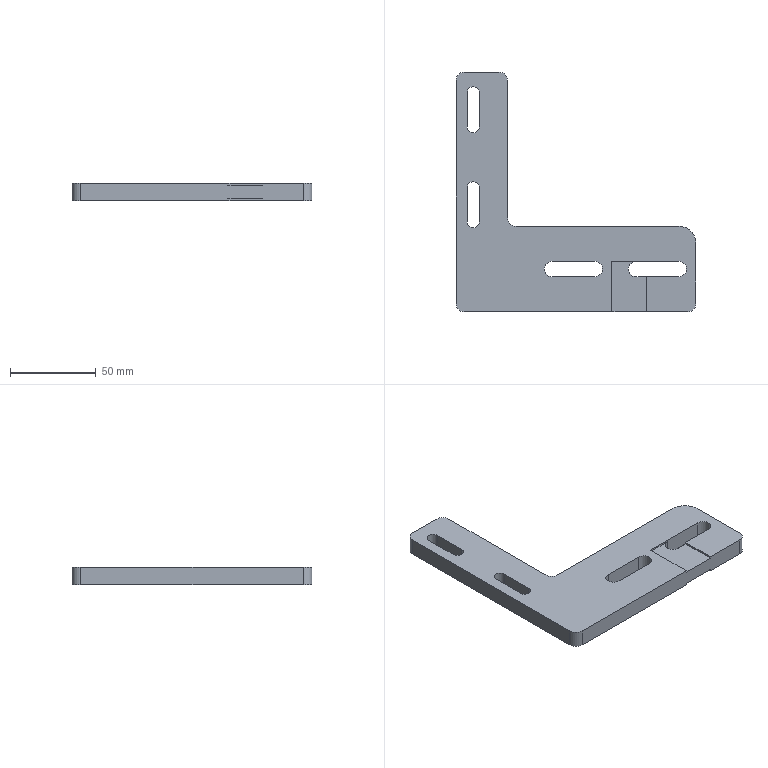Component | SolidWorks | Frame.1-1 | 1 solid | 38 faces | box 140 x 140 x 10 mm | volume 86274 mm3 | plane 22 | cylinder 16 | commonest cylinder face diameters 9 x6 10 x5 7 x4 20 x1
build123d program:
from build123d import *

# Parameters (mm, degrees)
BOSS_EXTRUDE1_DEPTH  = 10
CUT_EXTRUDE1_2_DEPTH = 1
CUT_EXTRUDE2_2_START = -1
CUT_EXTRUDE2_2_DEPTH = 1
SKETCH1_W            = 20
SKETCH1_H            = 7.5
CUT_EXTRUDE1_DEPTH   = 1
SKETCH2_W            = 20
SKETCH2_H            = 7.5
CUT_EXTRUDE2_DEPTH   = 1


with BuildPart() as part:
    # Sketch1_2 → Boss-Extrude1 (new body)
    with BuildSketch(Plane.XY):
        with BuildLine():
            Line((5, 0), (135, 0))
            ThreePointArc((135, 0), (138.536, 1.464), (140, 5))
            Line((140, 5), (140, 40))
            ThreePointArc((140, 40), (137.071, 47.071), (130, 50))
            Line((130, 50), (35, 50))
            ThreePointArc((35, 50), (31.464, 51.464), (30, 55))
            Line((30, 55), (30, 135))
            ThreePointArc((30, 135), (28.536, 138.536), (25, 140))
            Line((25, 140), (5, 140))
            ThreePointArc((5, 140), (1.464, 138.536), (0, 135))
            Line((0, 135), (0, 5))
            ThreePointArc((0, 5), (1.464, 1.464), (5, 0))
        make_face()
        with BuildLine():
            Line((105, 29.5), (130, 29.5))
            ThreePointArc((130, 29.5), (134.5, 25), (130, 20.5))
            Line((130, 20.5), (105, 20.5))
            ThreePointArc((105, 20.5), (100.5, 25), (105, 29.5))
        make_face(mode=Mode.SUBTRACT)
        with BuildLine():
            Line((56, 29.5), (81, 29.5))
            ThreePointArc((81, 29.5), (85.5, 25), (81, 20.5))
            Line((81, 20.5), (56, 20.5))
            ThreePointArc((56, 20.5), (51.5, 25), (56, 29.5))
        make_face(mode=Mode.SUBTRACT)
        with BuildLine():
            Line((13.5, 128), (13.5, 108))
            ThreePointArc((13.5, 108), (10, 104.5), (6.5, 108))
            Line((6.5, 108), (6.5, 128))
            ThreePointArc((6.5, 128), (10, 131.5), (13.5, 128))
        make_face(mode=Mode.SUBTRACT)
        with BuildLine():
            Line((13.5, 72.5), (13.5, 52.5))
            ThreePointArc((13.5, 52.5), (10, 49), (6.5, 52.5))
            Line((6.5, 52.5), (6.5, 72.5))
            ThreePointArc((6.5, 72.5), (10, 76), (13.5, 72.5))
        make_face(mode=Mode.SUBTRACT)
    extrude(amount=BOSS_EXTRUDE1_DEPTH)

    # Sketch2_2 → Cut-Extrude1_2 (cut)
    with BuildSketch(Plane(origin=(0, 0, 0), x_dir=(-1, 0, 0), z_dir=(0, 0, -1))):
        with BuildLine():
            Line((-111, 0), (-111, 25))
            Line((-111, 25), (-94, 25))
            ThreePointArc((-94, 25), (-91.879, 24.121), (-91, 22))
            Line((-91, 22), (-91, 0))
            Line((-91, 0), (-111, 0))
        make_face()
    extrude(amount=-CUT_EXTRUDE1_2_DEPTH, mode=Mode.SUBTRACT)

    # Sketch3 → Cut-Extrude2_2 (cut)
    with BuildSketch(Plane.XY.offset(10).offset(CUT_EXTRUDE2_2_START)):
        with BuildLine():
            Line((91, 0), (111, 0))
            Line((111, 0), (111, 25))
            Line((111, 25), (94, 25))
            ThreePointArc((94, 25), (91.879, 24.121), (91, 22))
            Line((91, 22), (91, 0))
        make_face()
    extrude(amount=CUT_EXTRUDE2_2_DEPTH, mode=Mode.SUBTRACT)

    # Sketch1 → Cut-Extrude1 (cut, symmetric)
    with BuildSketch(Plane(origin=(0, 0, 0), x_dir=(-1, 0, 0), z_dir=(0, 0, -1))):
        with Locations((-101, 25.75)):
            Rectangle(SKETCH1_W, SKETCH1_H)
    extrude(amount=CUT_EXTRUDE1_DEPTH, both=True, mode=Mode.SUBTRACT)

    # Sketch2 → Cut-Extrude2 (cut, symmetric)
    with BuildSketch(Plane.XY.offset(10)):
        with Locations((101, 25.75)):
            Rectangle(SKETCH2_W, SKETCH2_H)
    extrude(amount=CUT_EXTRUDE2_DEPTH, both=True, mode=Mode.SUBTRACT)


solid = part.part

# Placed as in the assembly
solid = solid.moved(Location((-60.5, 218, -89.4), (0, 0, 0)))